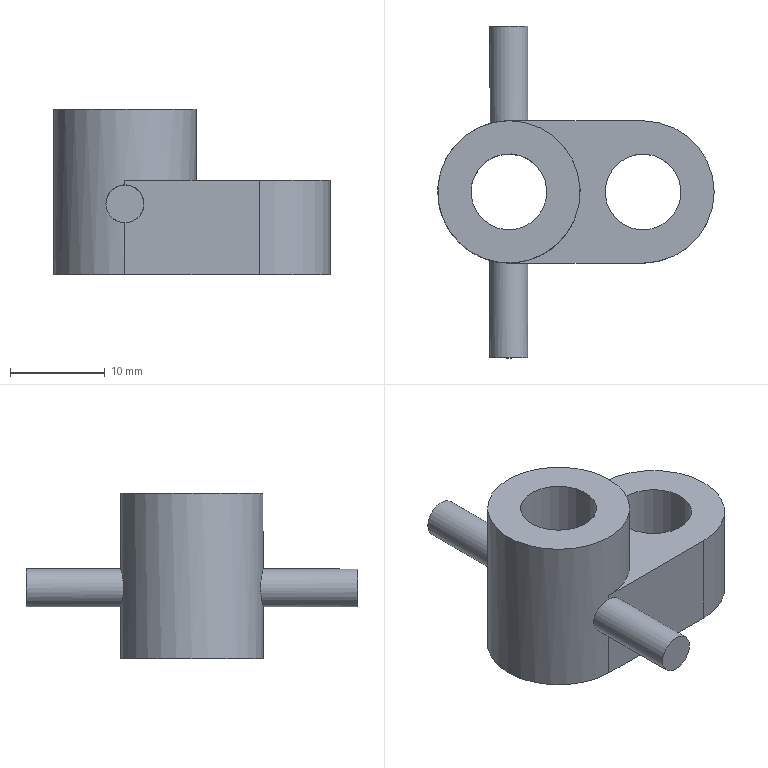Component | NX | STEERING_ROD | 1 solid | 13 faces | volume 4084 mm3 | plane 7 | cylinder 6 | commonest cylinder face diameters 15 x2 8 x2 4 x2